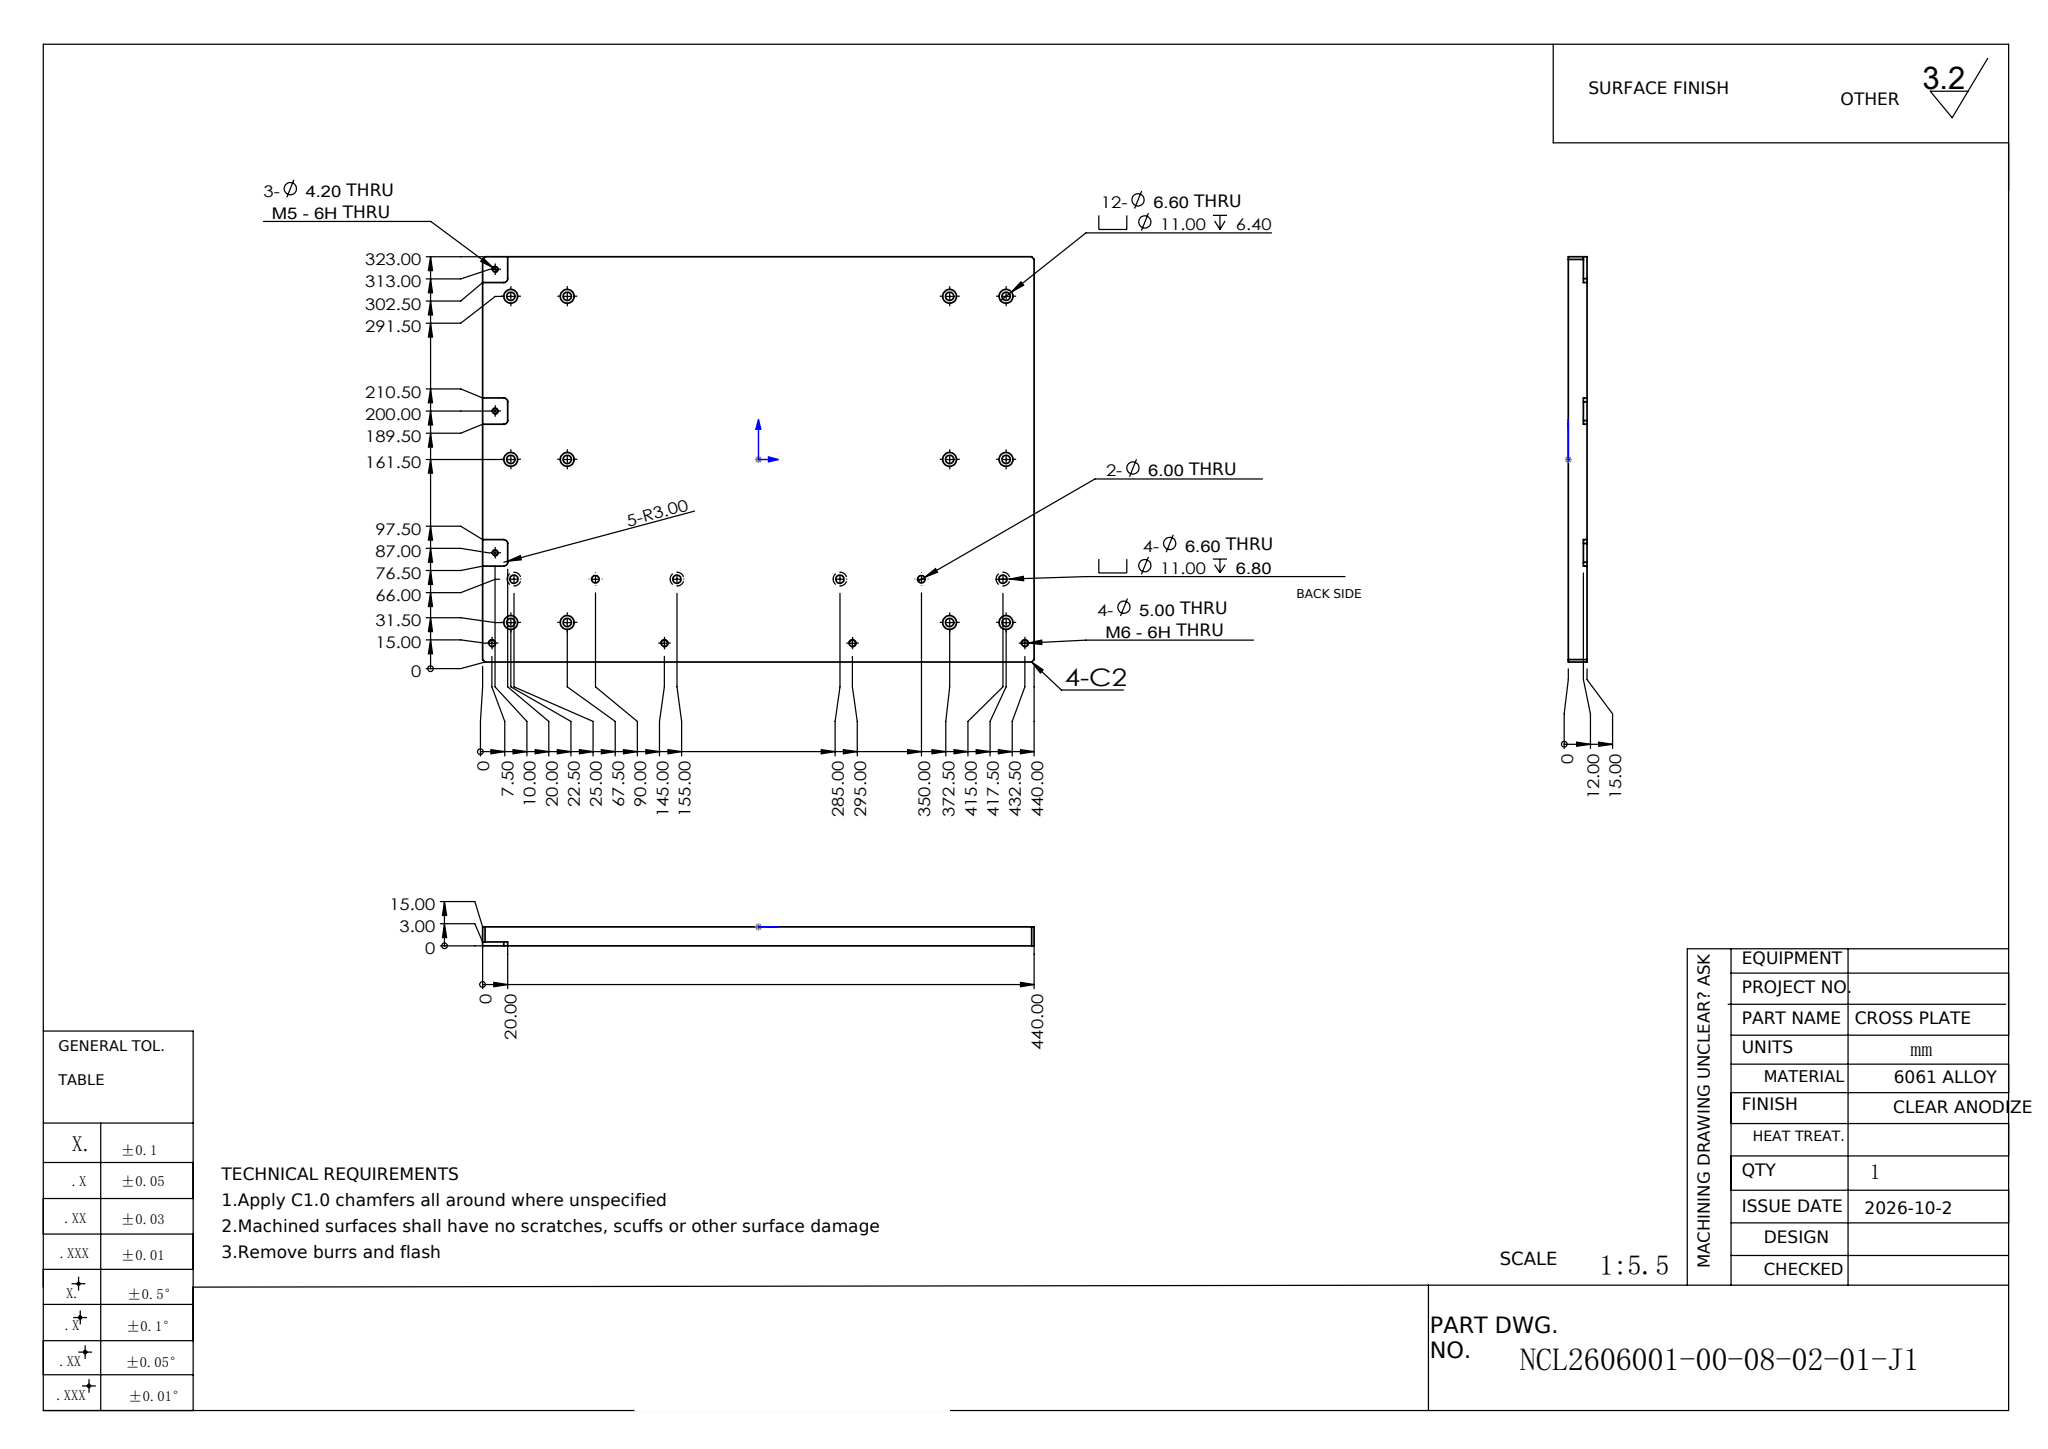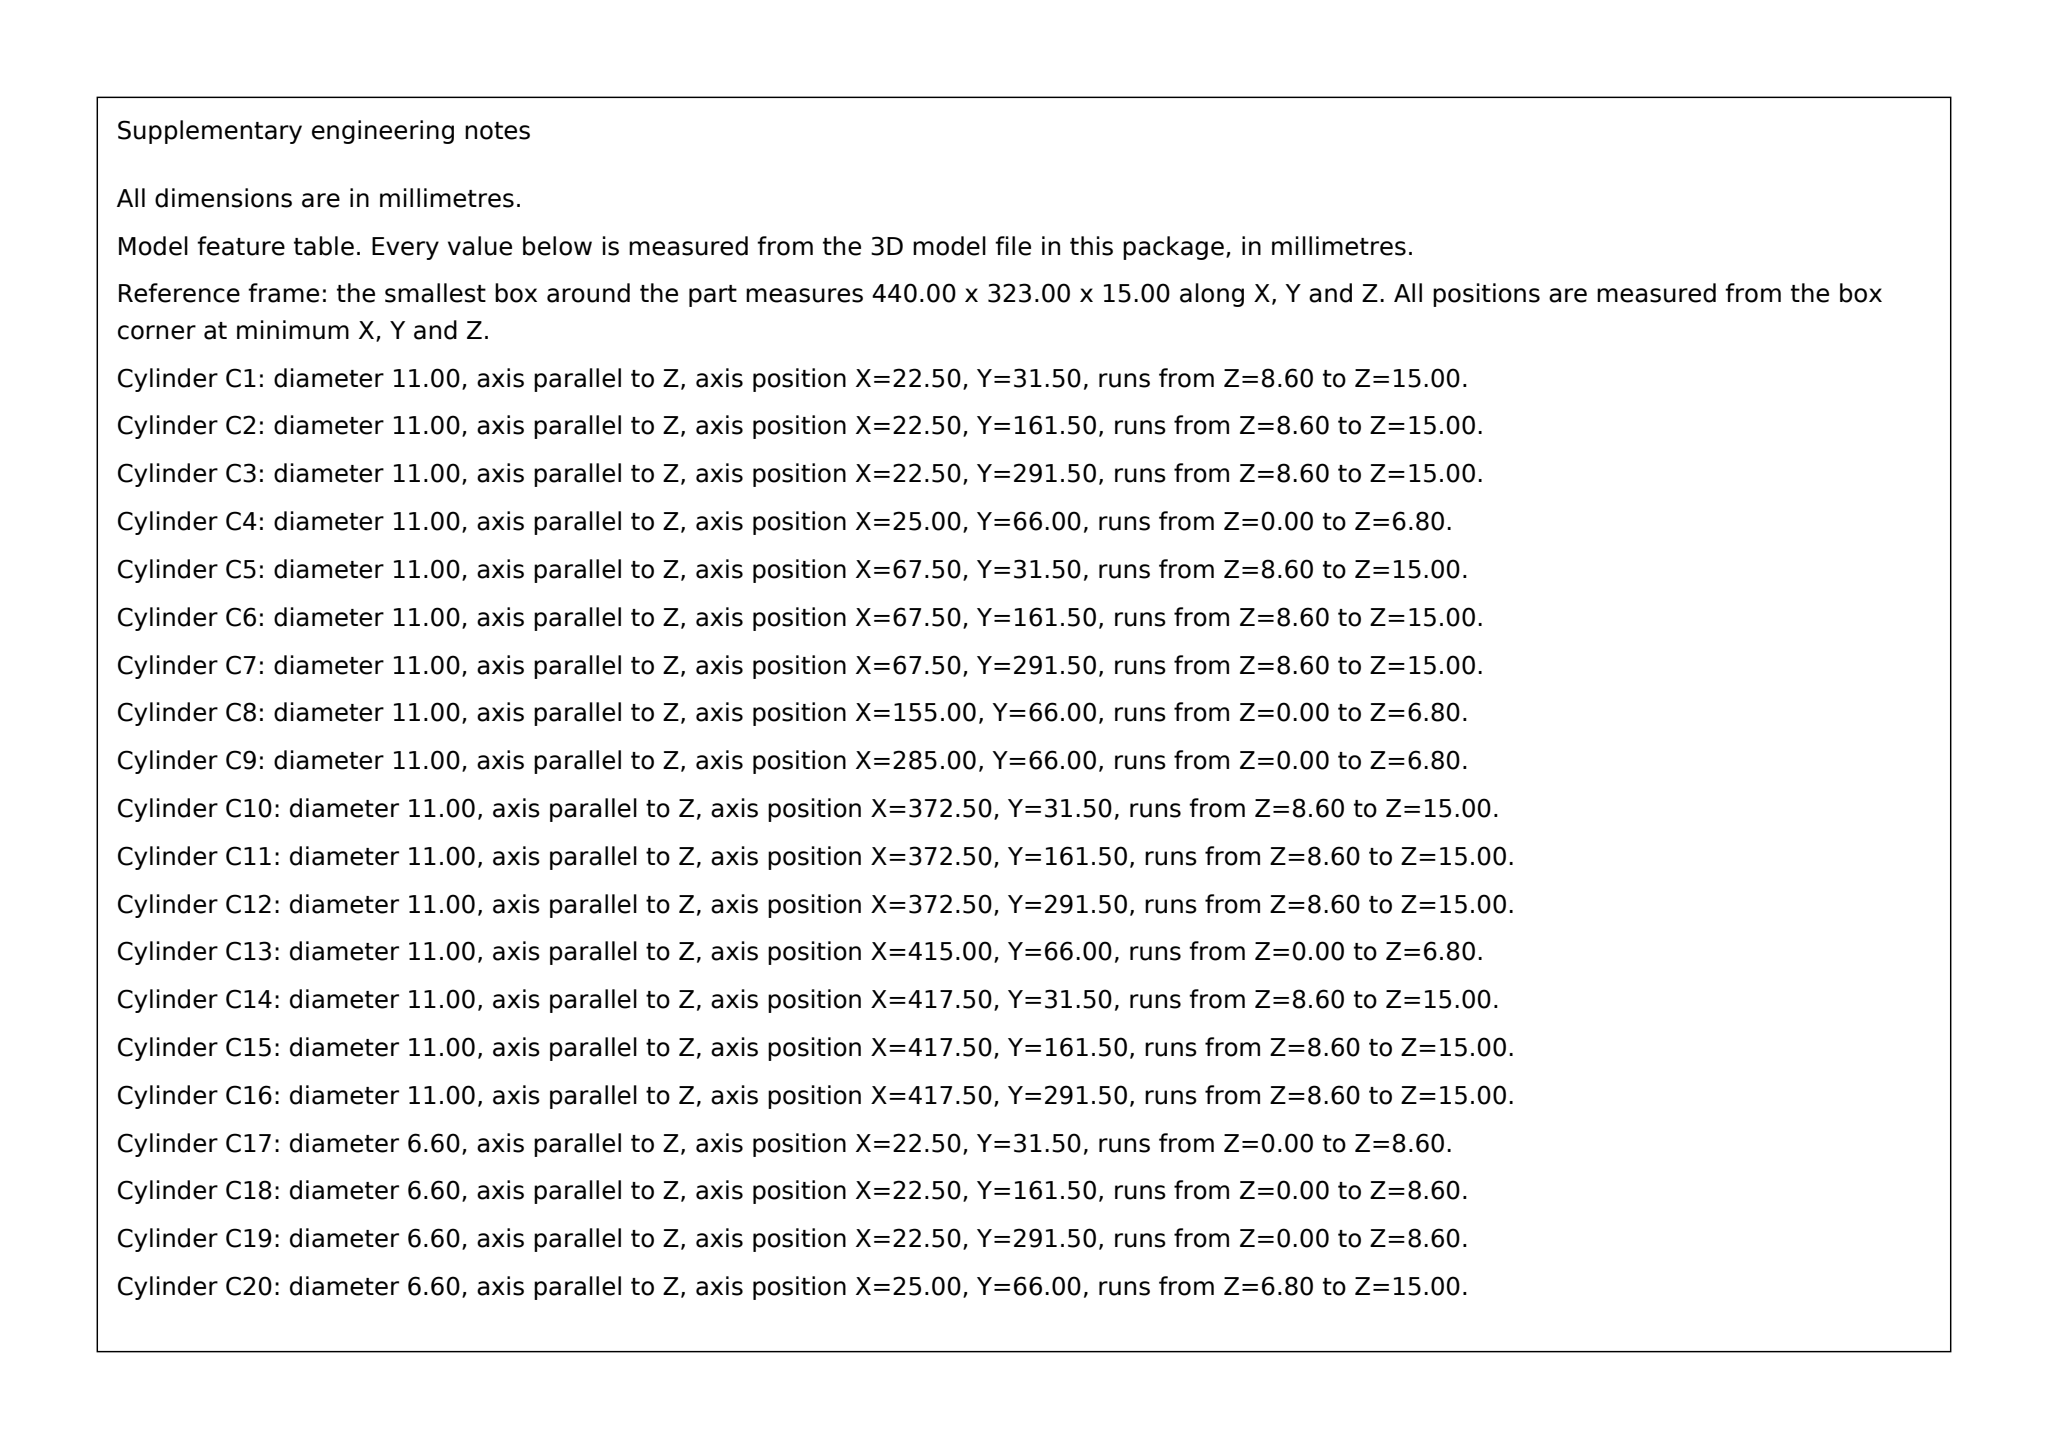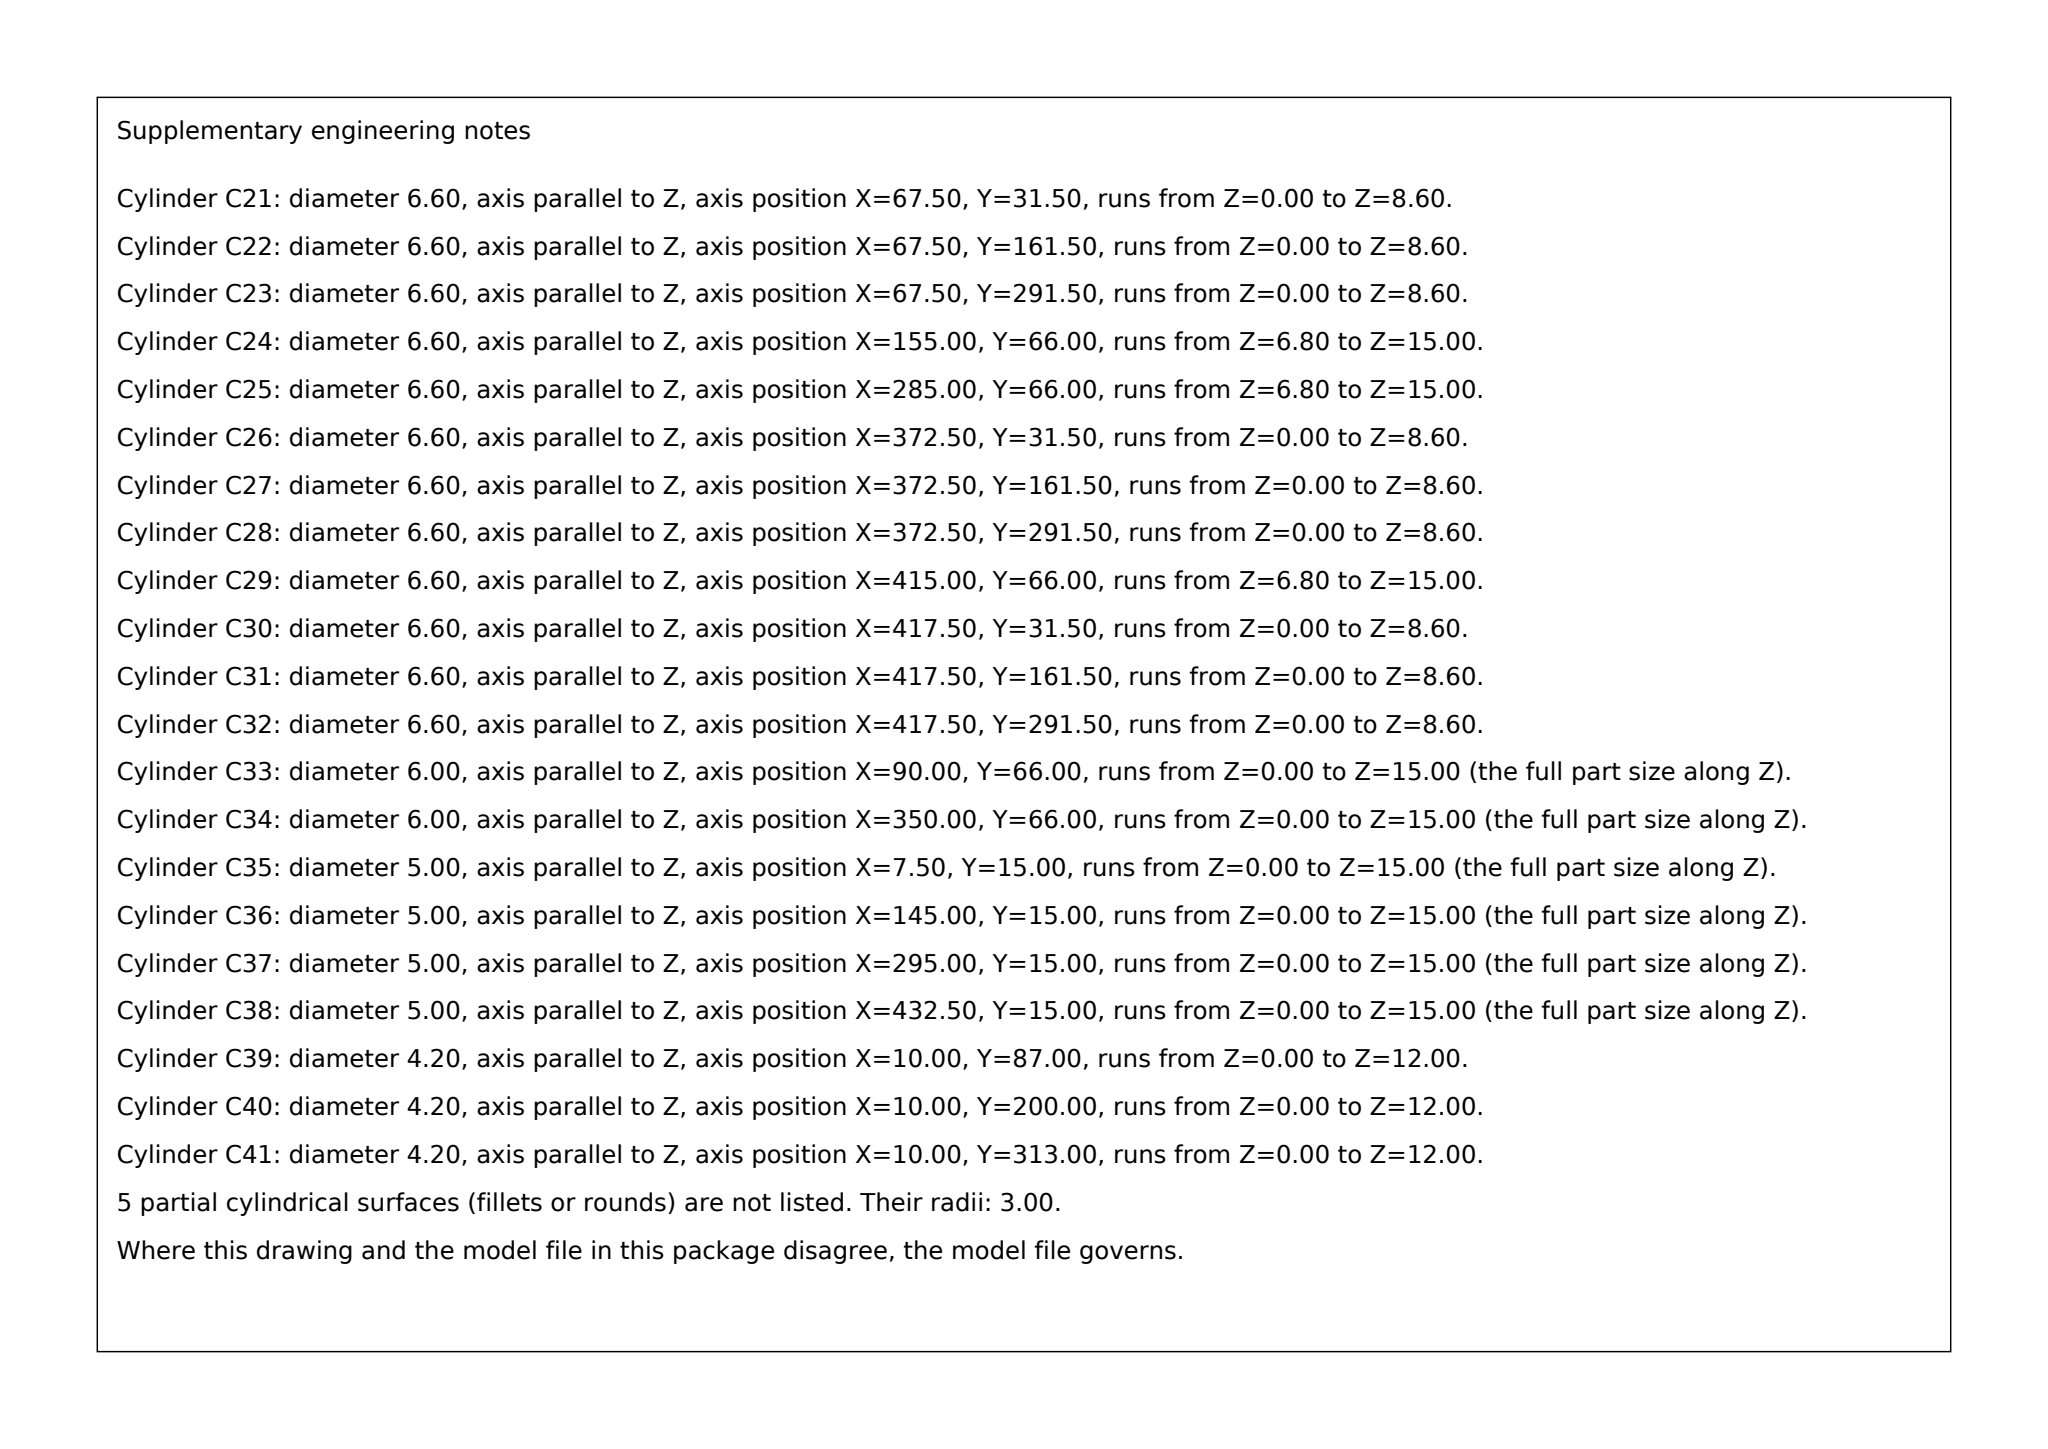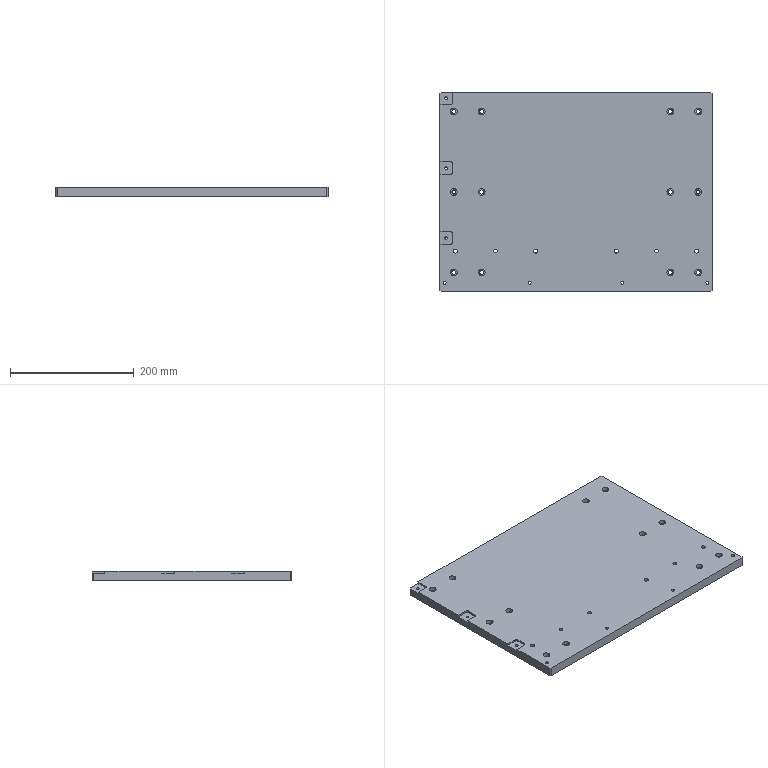Part | SolidWorks | mm | material 6061 ALLOY | 1 solid | 124 faces | box 440 x 323 x 15 mm | volume 2110904 mm3 | cylinder 87 | plane 37 | commonest cylinder face diameters 11 x32 6.6 x32 6 x9 5 x8 4.2 x6